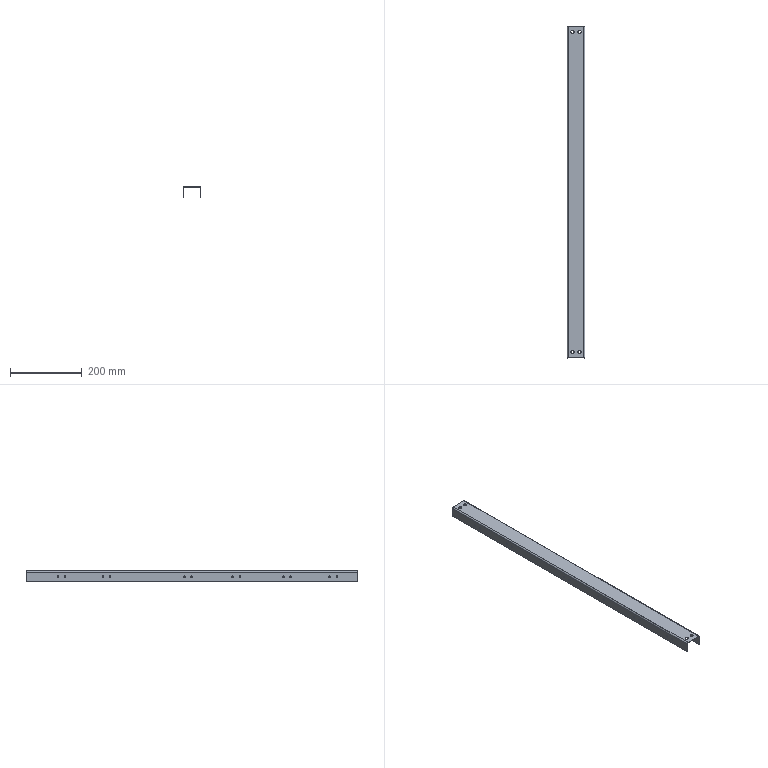Component | SolidWorks | FrameLongitudinalBeamSix100-2 | 1 solid | 82 faces | volume 143938 mm3 | cylinder 64 | plane 18 | commonest cylinder face diameters 4.5 x48 9 x8 6 x4 8 x2 5 x2